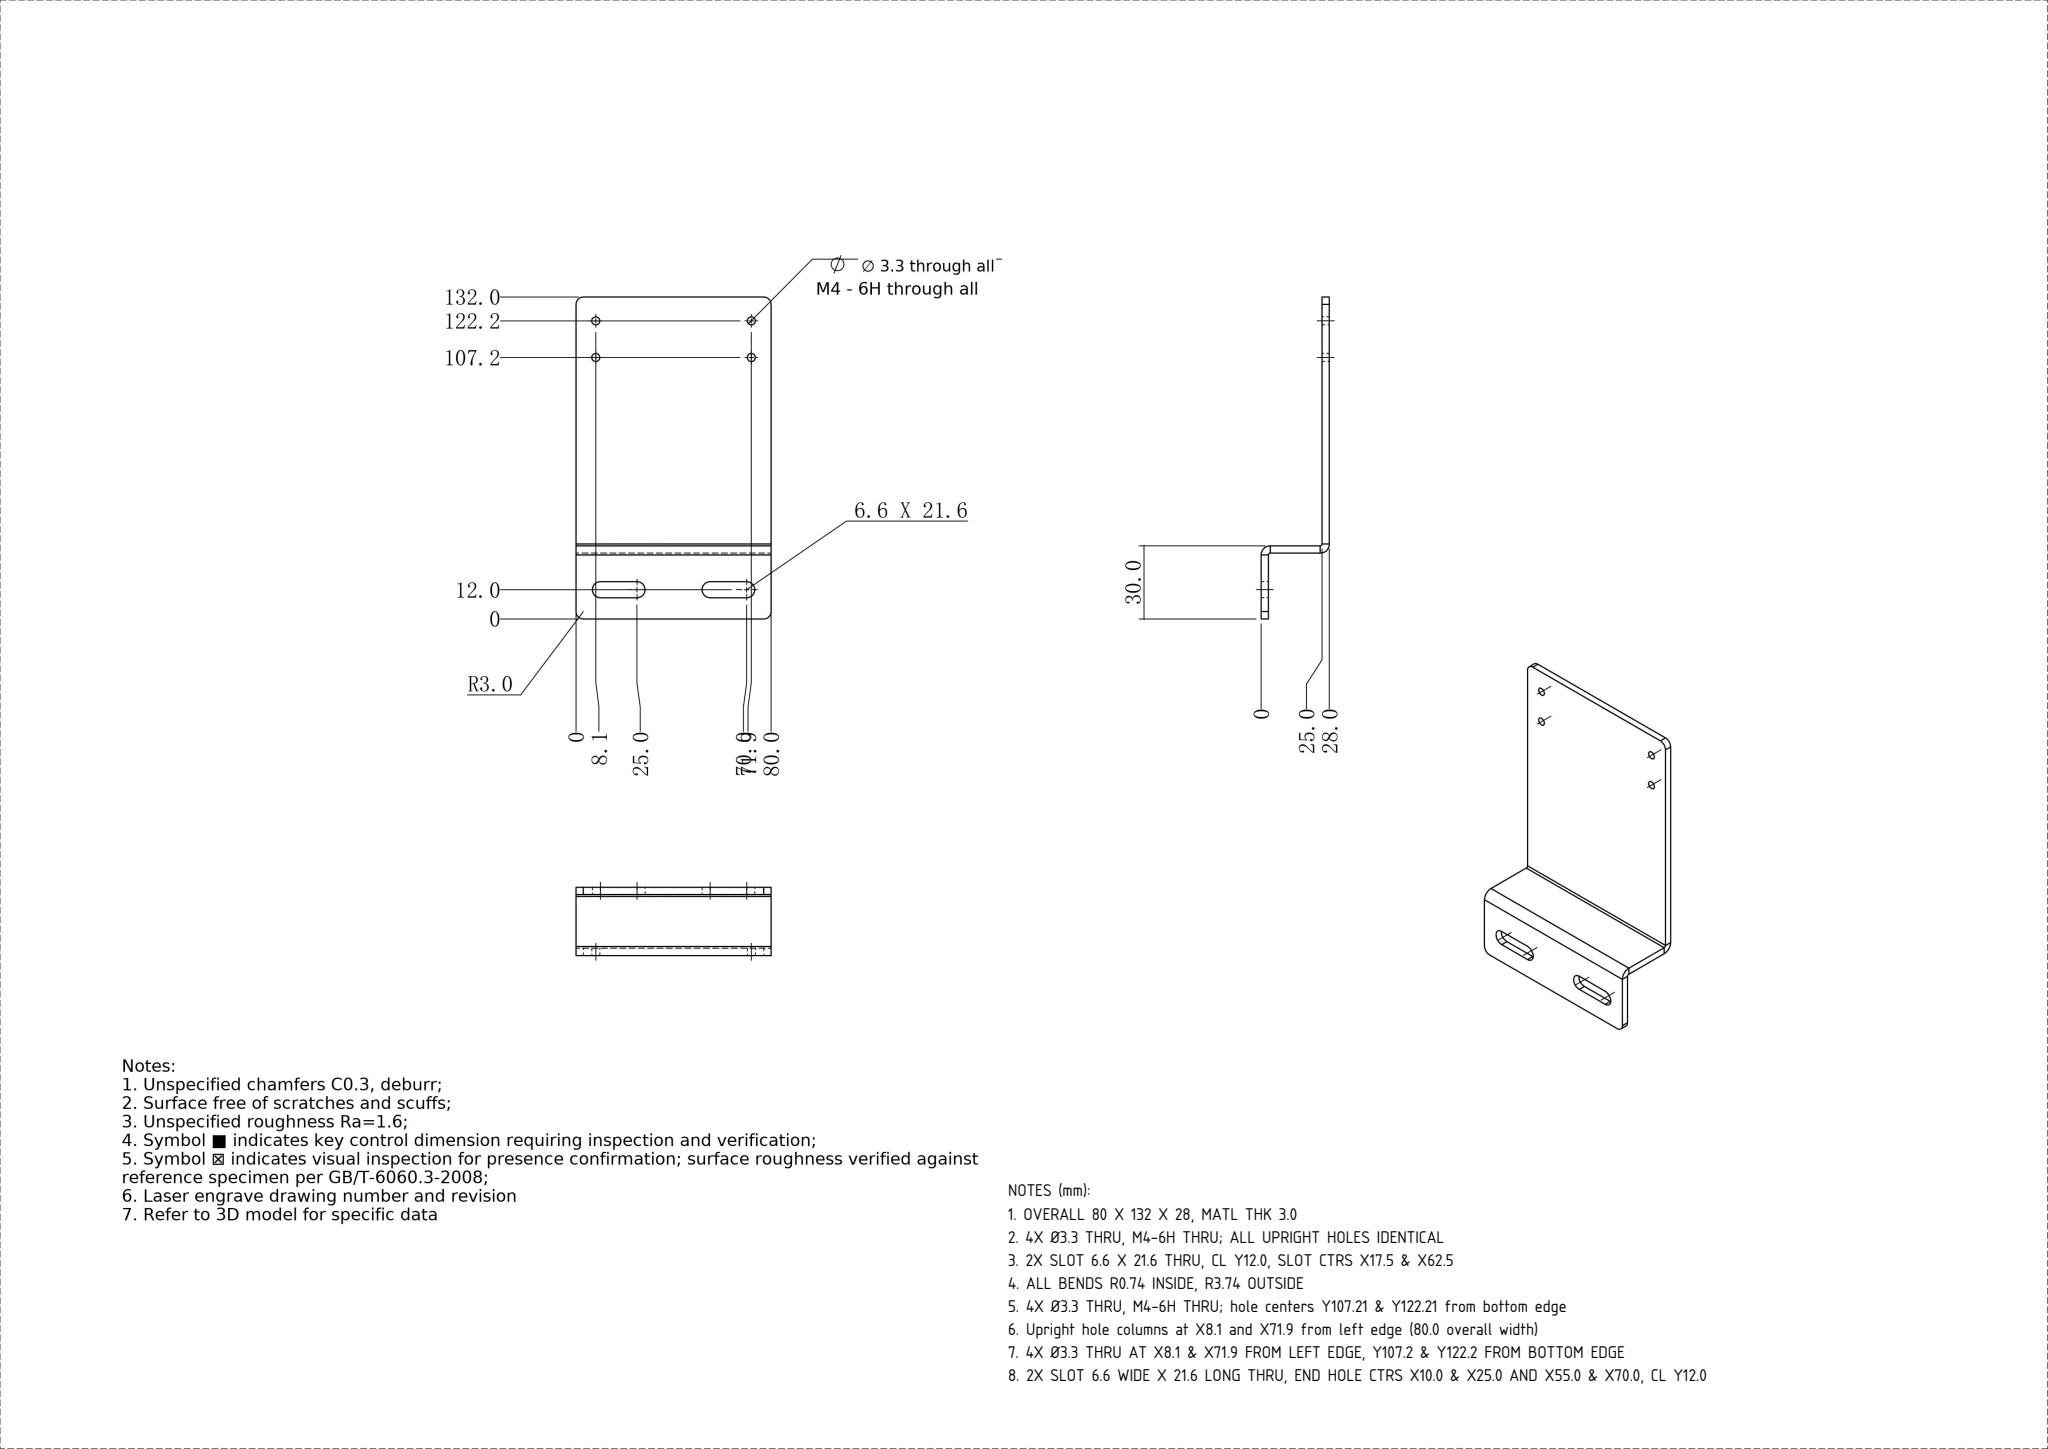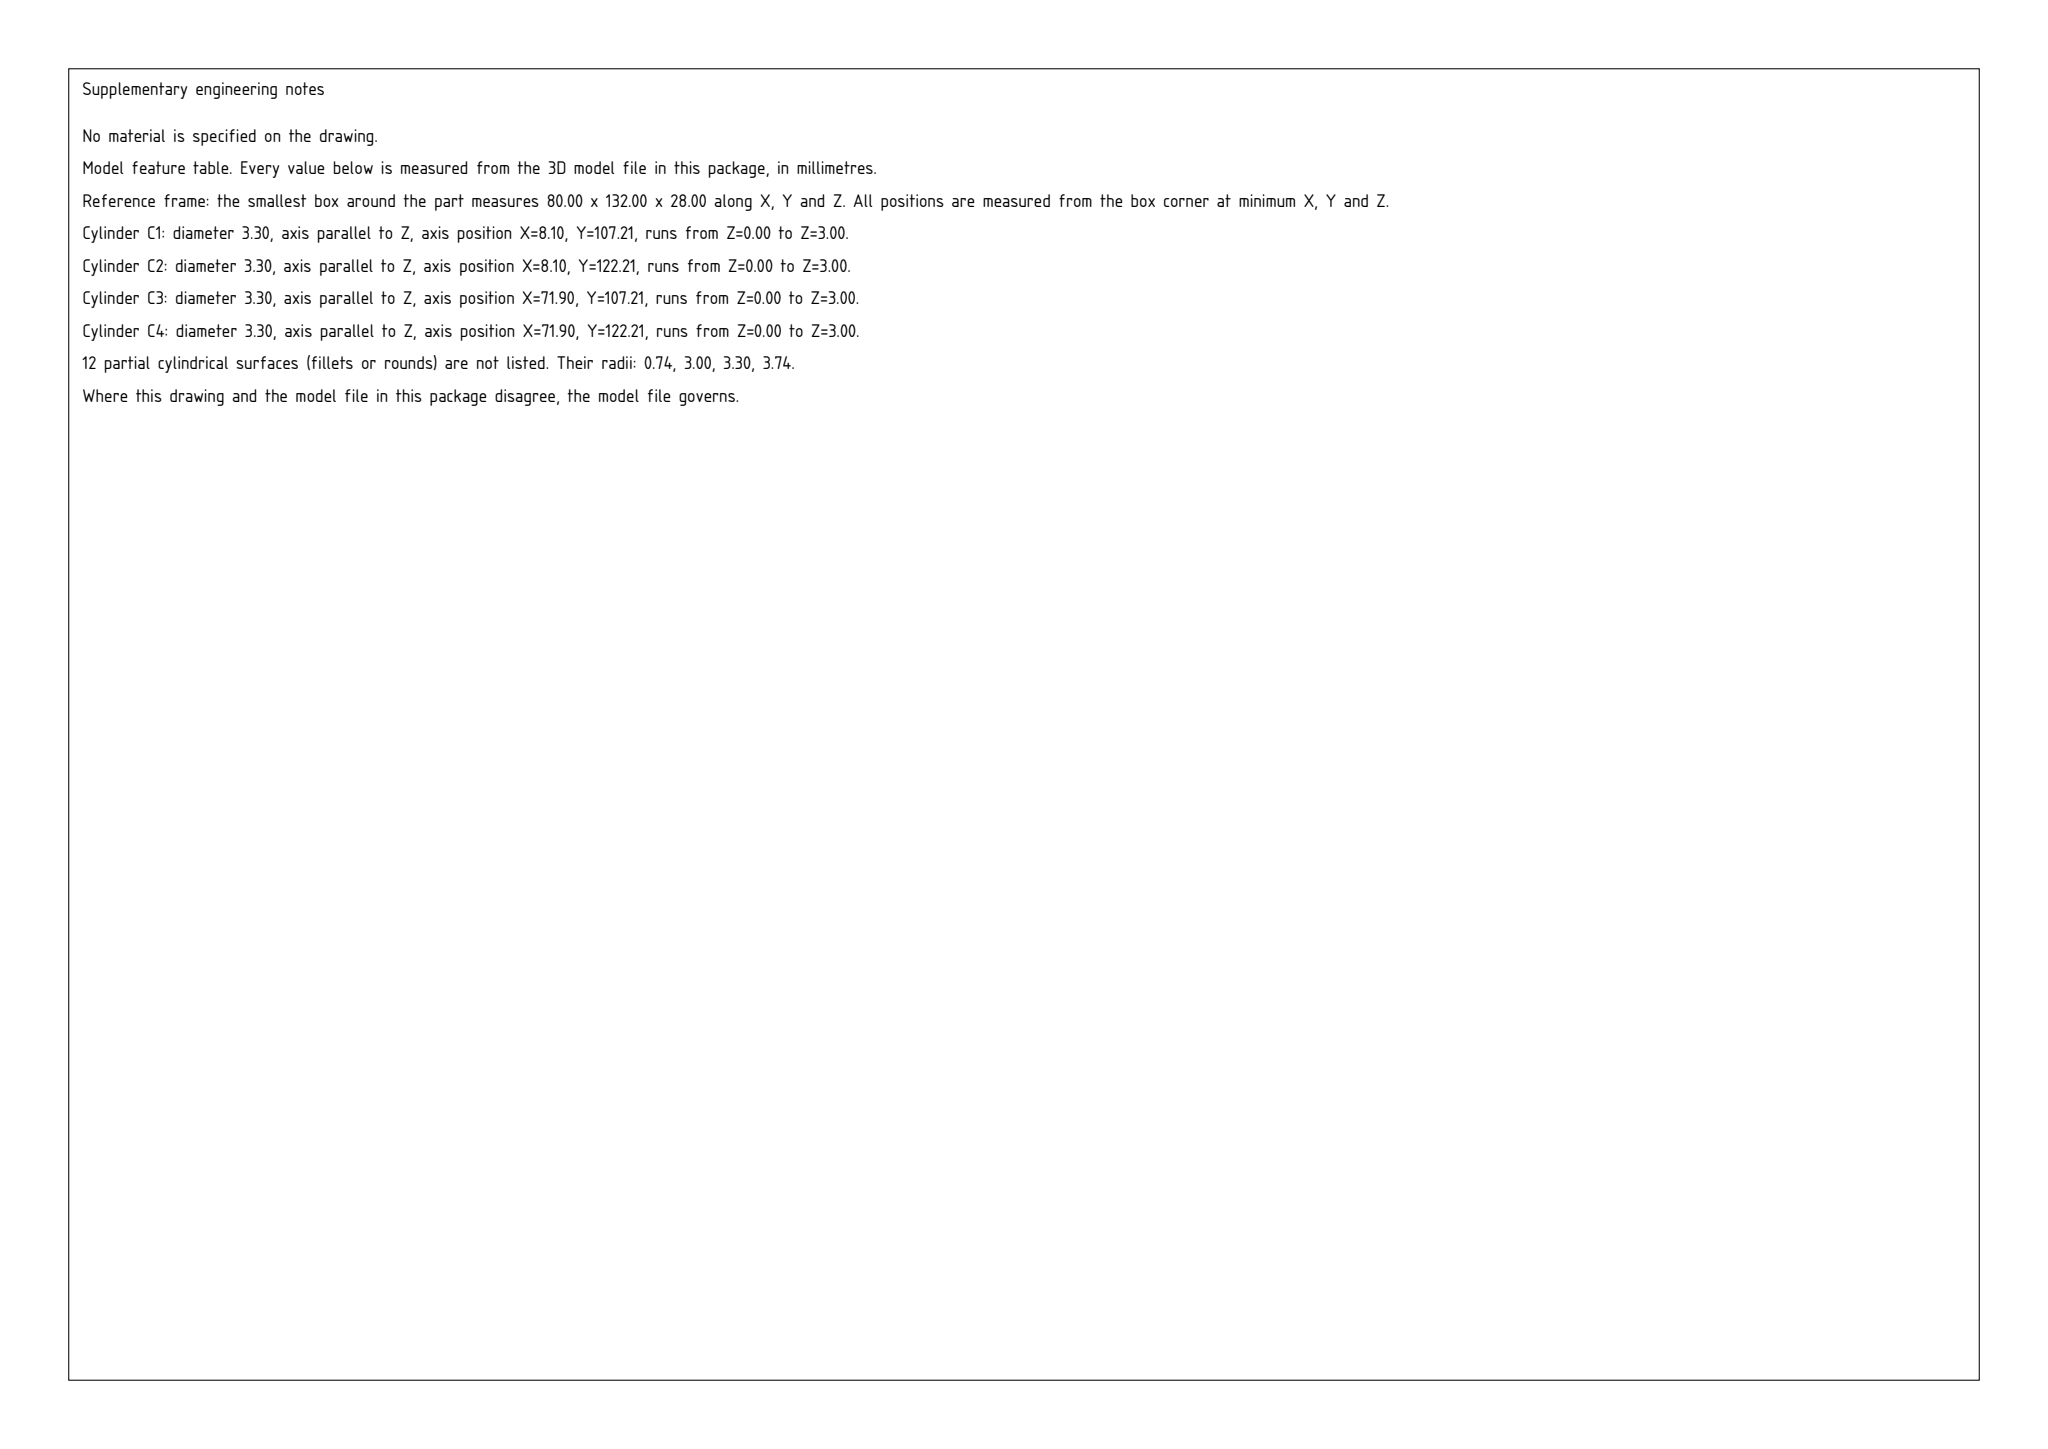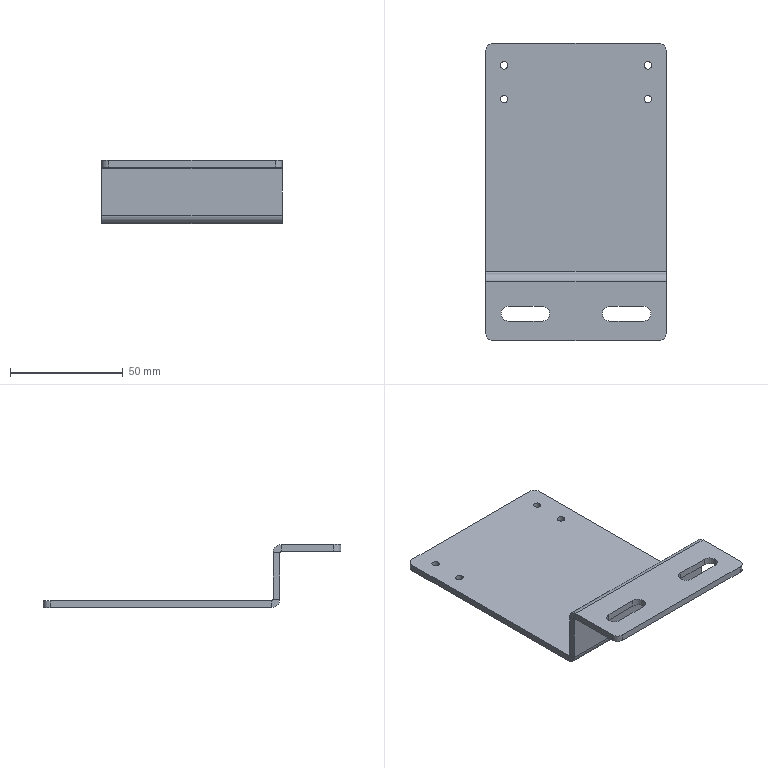Part | SolidWorks | mm | 1 solid | 42 faces | box 80 x 132 x 28 mm | volume 36294 mm3 | plane 22 | cylinder 20 | commonest cylinder face diameters 3.3 x8 6 x4 6.6 x4 7.473 x2 1.473 x2
Drawing notes:
OVERALL 80 X 132 X 28, MATL THK 3.0 | from the solid: bbox 80x132x28; wall z0-3 and y27-30 gives 3.0 thk
4X Ø3.3 THRU, M4-6H THRU; ALL UPRIGHT HOLES IDENTICAL | from the solid: Four Ø3.3 z-axis holes at x=8.1/71.9, y=107.21/122.21; no other hole dia present
2X SLOT 6.6 X 21.6 THRU, CL Y12.0, SLOT CTRS X17.5 & X62.5 | from the solid: Ø6.6 end cyls at x=10/25 and x=55/70, y=12.0; 15+6.6=21.6 long
ALL BENDS R0.74 INSIDE, R3.74 OUTSIDE | from the solid: x-axis cyls Ø1.473 (R0.737) & Ø7.473 (R3.737) at y26.26/z24.26 and y30.74/z3.74
4X Ø3.3 THRU, M4-6H THRU; hole centers Y107.21 & Y122.21 from bottom edge | from the solid: cylinders dia 3.3, axis z, length 3.0 at (8.1,107.21), (8.1,122.21), (71.9,107.21), (71.9,122.21)
Upright hole columns at X8.1 and X71.9 from left edge (80.0 overall width) | from the solid: cylinders dia 3.3, axis z, pos x = 8.1 and 71.9; bbox_xyz X = 80.0
4X Ø3.3 THRU AT X8.1 & X71.9 FROM LEFT EDGE, Y107.2 & Y122.2 FROM BOTTOM EDGE | from the solid: cylinders dia 3.3 axis z at (8.1,107.21), (8.1,122.21), (71.9,107.21), (71.9,122.21), length 3.0
2X SLOT 6.6 WIDE X 21.6 LONG THRU, END HOLE CTRS X10.0 & X25.0 AND X55.0 & X70.0, CL Y12.0 | from the solid: cylinders dia 6.6 axis z at (10.0,12.0), (25.0,12.0), (55.0,12.0), (70.0,12.0), length 3.0